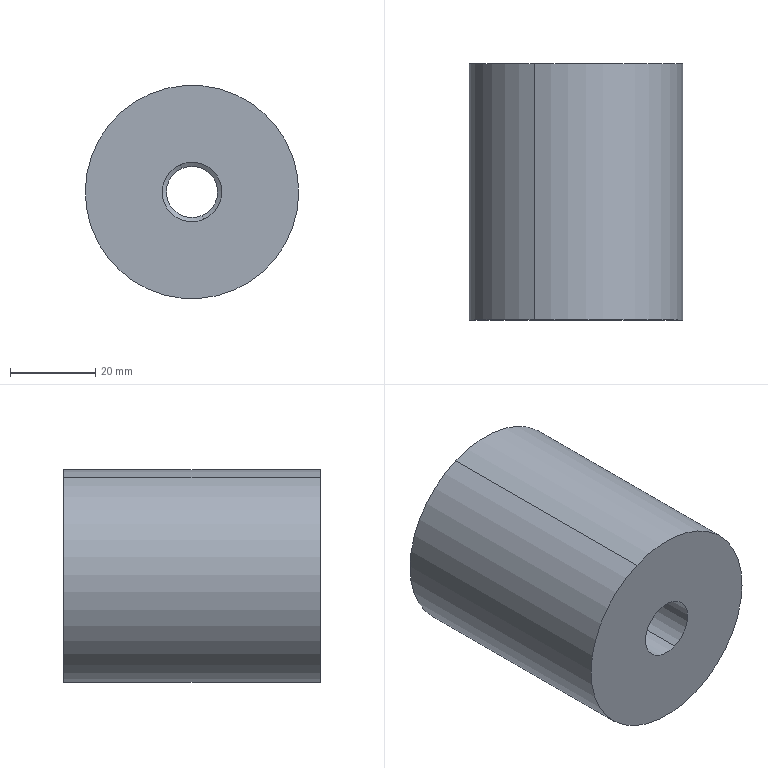Component | SolidWorks | KSD171005A-01-01-22-1 | 1 solid | 10 faces | box 50 x 60 x 50 mm | volume 109378 mm3 | cylinder 6 | cone 2 | plane 2 | commonest cylinder face diameters 14 x2 12 x2 50 x2
build123d program:
from build123d import *

# Parameters (mm, degrees)
SKETCH1_R                      = 25
BOSS_EXTRUDE1_DEPTH            = 60
M12_TAPPED_HOLE1_D             = 12
F_14_0_14_DIAMETER_HOLE1_D     = 14
F_14_0_14_DIAMETER_HOLE1_DEPTH = 40
F_14_0_14_DIAMETER_HOLE1_TIP   = 4.206


with BuildPart() as part:
    # Sketch1 → Boss-Extrude1 (new body)
    with BuildSketch(Plane.XY):
        Circle(SKETCH1_R)
    extrude(amount=BOSS_EXTRUDE1_DEPTH)

    # M12 Tapped Hole1 (through all)
    with Locations(Plane.XY.offset(60)):
        with Locations((0, 0)):
            Hole(M12_TAPPED_HOLE1_D / 2)

    # 14.0 _14_ Diameter Hole1
    with Locations(Plane.XY.offset(60)):
        with Locations((0, 0)):
            Hole(F_14_0_14_DIAMETER_HOLE1_D / 2, depth=F_14_0_14_DIAMETER_HOLE1_DEPTH)
            with Locations((0, 0, -(F_14_0_14_DIAMETER_HOLE1_DEPTH + F_14_0_14_DIAMETER_HOLE1_TIP / 2))):  # 118° drill point
                Cone(0, F_14_0_14_DIAMETER_HOLE1_D / 2, F_14_0_14_DIAMETER_HOLE1_TIP, mode=Mode.SUBTRACT)


solid = part.part

# Placed as in the assembly
solid = solid.moved(Location((-7.111, 170.73, 407), (90, 0, 0)))
STEP:
#1=COLOUR_RGB('',0.7922,0.8196,0.9333);
#2=FILL_AREA_STYLE_COLOUR('',#1);
#3=FILL_AREA_STYLE('',(#2));
#4=SURFACE_STYLE_FILL_AREA(#3);
#5=SURFACE_SIDE_STYLE('',(#4));
#6=SURFACE_STYLE_USAGE(.BOTH.,#5);
#7=PRESENTATION_STYLE_ASSIGNMENT((#6));
#8=CARTESIAN_POINT('',(-0.388,5.934,16.277));
#9=VERTEX_POINT('',#8);
#10=CARTESIAN_POINT('',(-0.172,5.934,15.77));
#11=VERTEX_POINT('',#10);
#12=CARTESIAN_POINT('',(-0.28,5.934,16.024));
#13=DIRECTION('',(0.,-1.,-0.));
#14=DIRECTION('',(0.3918,0.,-0.92));
#15=AXIS2_PLACEMENT_3D('',#12,#13,#14);
#16=CIRCLE('',#15,0.2756);
#17=EDGE_CURVE('',#9,#11,#16,.T.);
#18=ORIENTED_EDGE('',*,*,#17,.F.);
#19=CARTESIAN_POINT('',(-0.388,4.359,16.277));
#20=VERTEX_POINT('',#19);
#21=CARTESIAN_POINT('',(-0.388,4.359,16.277));
#22=DIRECTION('',(0.,-1.,-0.));
#23=VECTOR('',#22,39.37);
#24=LINE('',#21,#23);
#25=EDGE_CURVE('',#9,#20,#24,.T.);
#26=ORIENTED_EDGE('',*,*,#25,.T.);
#27=CARTESIAN_POINT('',(-0.172,4.359,15.77));
#28=VERTEX_POINT('',#27);
#29=CARTESIAN_POINT('',(-0.28,4.359,16.024));
#30=DIRECTION('',(0.,-1.,-0.));
#31=DIRECTION('',(0.3918,0.,-0.92));
#32=AXIS2_PLACEMENT_3D('',#29,#30,#31);
#33=CIRCLE('',#32,0.2756);
#34=EDGE_CURVE('',#20,#28,#33,.T.);
#35=ORIENTED_EDGE('',*,*,#34,.T.);
#36=CARTESIAN_POINT('',(-0.172,4.359,15.77));
#37=DIRECTION('',(0.,-1.,-0.));
#38=VECTOR('',#37,39.37);
#39=LINE('',#36,#38);
#40=EDGE_CURVE('',#11,#28,#39,.T.);
#41=ORIENTED_EDGE('',*,*,#40,.F.);
#42=EDGE_LOOP('',(#18,#26,#35,#41));
#43=FACE_OUTER_BOUND('',#42,.T.);
#44=CARTESIAN_POINT('',(-0.28,4.359,16.024));
#45=DIRECTION('',(0.,-1.,-0.));
#46=DIRECTION('',(0.3918,0.,-0.92));
#47=AXIS2_PLACEMENT_3D('',#44,#45,#46);
#48=CYLINDRICAL_SURFACE('',#47,0.2756);
#49=ADVANCED_FACE('',(#43),#48,.F.);
#50=CARTESIAN_POINT('',(-0.3725,5.958,16.241));
#51=VERTEX_POINT('',#50);
#52=CARTESIAN_POINT('',(-0.1874,5.958,15.806));
#53=VERTEX_POINT('',#52);
#54=CARTESIAN_POINT('',(-0.28,5.958,16.024));
#55=DIRECTION('',(0.,-1.,-0.));
#56=DIRECTION('',(0.3918,0.,-0.92));
#57=AXIS2_PLACEMENT_3D('',#54,#55,#56);
#58=CIRCLE('',#57,0.2362);
#59=EDGE_CURVE('',#51,#53,#58,.T.);
#60=ORIENTED_EDGE('',*,*,#59,.F.);
#61=CARTESIAN_POINT('',(-0.388,5.934,16.277));
#62=DIRECTION('',(-0.3359,-0.515,0.7886));
#63=VECTOR('',#62,39.37);
#64=LINE('',#61,#63);
#65=EDGE_CURVE('',#51,#9,#64,.T.);
#66=ORIENTED_EDGE('',*,*,#65,.T.);
#67=ORIENTED_EDGE('',*,*,#17,.T.);
#68=CARTESIAN_POINT('',(-0.172,5.934,15.77));
#69=DIRECTION('',(0.3359,-0.515,-0.7886));
#70=VECTOR('',#69,39.37);
#71=LINE('',#68,#70);
#72=EDGE_CURVE('',#53,#11,#71,.T.);
#73=ORIENTED_EDGE('',*,*,#72,.F.);
#74=EDGE_LOOP('',(#60,#66,#67,#73));
#75=FACE_OUTER_BOUND('',#74,.T.);
#76=CARTESIAN_POINT('',(-0.28,5.934,16.024));
#77=DIRECTION('',(0.,-1.,-0.));
#78=DIRECTION('',(0.3918,0.,-0.92));
#79=AXIS2_PLACEMENT_3D('',#76,#77,#78);
#80=CONICAL_SURFACE('',#79,0.2756,1.03);
#81=ADVANCED_FACE('',(#75),#80,.F.);
#82=CARTESIAN_POINT('',(-0.3725,6.722,16.241));
#83=VERTEX_POINT('',#82);
#84=CARTESIAN_POINT('',(-0.1874,6.722,15.806));
#85=VERTEX_POINT('',#84);
#86=CARTESIAN_POINT('',(-0.28,6.722,16.024));
#87=DIRECTION('',(0.,-1.,-0.));
#88=DIRECTION('',(0.3918,0.,-0.92));
#89=AXIS2_PLACEMENT_3D('',#86,#87,#88);
#90=CIRCLE('',#89,0.2362);
#91=EDGE_CURVE('',#83,#85,#90,.T.);
#92=ORIENTED_EDGE('',*,*,#91,.F.);
#93=CARTESIAN_POINT('',(-0.3725,4.359,16.241));
#94=DIRECTION('',(0.,-1.,-0.));
#95=VECTOR('',#94,39.37);
#96=LINE('',#93,#95);
#97=EDGE_CURVE('',#83,#51,#96,.T.);
#98=ORIENTED_EDGE('',*,*,#97,.T.);
#99=ORIENTED_EDGE('',*,*,#59,.T.);
#100=CARTESIAN_POINT('',(-0.1874,4.359,15.806));
#101=DIRECTION('',(0.,-1.,-0.));
#102=VECTOR('',#101,39.37);
#103=LINE('',#100,#102);
#104=EDGE_CURVE('',#85,#53,#103,.T.);
#105=ORIENTED_EDGE('',*,*,#104,.F.);
#106=EDGE_LOOP('',(#92,#98,#99,#105));
#107=FACE_OUTER_BOUND('',#106,.T.);
#108=CARTESIAN_POINT('',(-0.28,4.359,16.024));
#109=DIRECTION('',(0.,-1.,-0.));
#110=DIRECTION('',(0.3918,0.,-0.92));
#111=AXIS2_PLACEMENT_3D('',#108,#109,#110);
#112=CYLINDRICAL_SURFACE('',#111,0.2362);
#113=ADVANCED_FACE('',(#107),#112,.F.);
#114=CARTESIAN_POINT('',(0.1057,4.359,15.118));
#115=VERTEX_POINT('',#114);
#116=CARTESIAN_POINT('',(-0.6656,4.359,16.929));
#117=VERTEX_POINT('',#116);
#118=CARTESIAN_POINT('',(-0.28,4.359,16.024));
#119=DIRECTION('',(0.,-1.,-0.));
#120=DIRECTION('',(0.3918,0.,-0.92));
#121=AXIS2_PLACEMENT_3D('',#118,#119,#120);
#122=CIRCLE('',#121,0.9843);
#123=EDGE_CURVE('',#115,#117,#122,.T.);
#124=ORIENTED_EDGE('',*,*,#123,.F.);
#125=CARTESIAN_POINT('',(0.1057,6.722,15.118));
#126=VERTEX_POINT('',#125);
#127=CARTESIAN_POINT('',(0.1057,4.359,15.118));
#128=DIRECTION('',(-0.,1.,0.));
#129=VECTOR('',#128,39.37);
#130=LINE('',#127,#129);
#131=EDGE_CURVE('',#115,#126,#130,.T.);
#132=ORIENTED_EDGE('',*,*,#131,.T.);
#133=CARTESIAN_POINT('',(-0.6656,6.722,16.929));
#134=VERTEX_POINT('',#133);
#135=CARTESIAN_POINT('',(-0.28,6.722,16.024));
#136=DIRECTION('',(0.,-1.,-0.));
#137=DIRECTION('',(0.3918,0.,-0.92));
#138=AXIS2_PLACEMENT_3D('',#135,#136,#137);
#139=CIRCLE('',#138,0.9843);
#140=EDGE_CURVE('',#126,#134,#139,.T.);
#141=ORIENTED_EDGE('',*,*,#140,.T.);
#142=CARTESIAN_POINT('',(-0.6656,4.359,16.929));
#143=DIRECTION('',(-0.,1.,0.));
#144=VECTOR('',#143,39.37);
#145=LINE('',#142,#144);
#146=EDGE_CURVE('',#117,#134,#145,.T.);
#147=ORIENTED_EDGE('',*,*,#146,.F.);
#148=EDGE_LOOP('',(#124,#132,#141,#147));
#149=FACE_OUTER_BOUND('',#148,.T.);
#150=CARTESIAN_POINT('',(-0.28,4.359,16.024));
#151=DIRECTION('',(-0.,1.,0.));
#152=DIRECTION('',(-0.3918,0.,0.92));
#153=AXIS2_PLACEMENT_3D('',#150,#151,#152);
#154=CYLINDRICAL_SURFACE('',#153,0.9843);
#155=ADVANCED_FACE('',(#149),#154,.T.);
#156=ORIENTED_EDGE('',*,*,#131,.F.);
#157=CARTESIAN_POINT('',(-0.28,4.359,16.024));
#158=DIRECTION('',(0.,-1.,-0.));
#159=DIRECTION('',(0.3918,0.,-0.92));
#160=AXIS2_PLACEMENT_3D('',#157,#158,#159);
#161=CIRCLE('',#160,0.9843);
#162=EDGE_CURVE('',#117,#115,#161,.T.);
#163=ORIENTED_EDGE('',*,*,#162,.F.);
#164=ORIENTED_EDGE('',*,*,#146,.T.);
#165=CARTESIAN_POINT('',(-0.28,6.722,16.024));
#166=DIRECTION('',(0.,-1.,-0.));
#167=DIRECTION('',(0.3918,0.,-0.92));
#168=AXIS2_PLACEMENT_3D('',#165,#166,#167);
#169=CIRCLE('',#168,0.9843);
#170=EDGE_CURVE('',#134,#126,#169,.T.);
#171=ORIENTED_EDGE('',*,*,#170,.T.);
#172=EDGE_LOOP('',(#156,#163,#164,#171));
#173=FACE_OUTER_BOUND('',#172,.T.);
#174=CARTESIAN_POINT('',(-0.28,4.359,16.024));
#175=DIRECTION('',(-0.,1.,0.));
#176=DIRECTION('',(-0.3918,0.,0.92));
#177=AXIS2_PLACEMENT_3D('',#174,#175,#176);
#178=CYLINDRICAL_SURFACE('',#177,0.9843);
#179=ADVANCED_FACE('',(#173),#178,.T.);
#180=CARTESIAN_POINT('',(-0.28,4.359,16.024));
#181=DIRECTION('',(0.,-1.,-0.));
#182=DIRECTION('',(0.3918,0.,-0.92));
#183=AXIS2_PLACEMENT_3D('',#180,#181,#182);
#184=CIRCLE('',#183,0.2756);
#185=EDGE_CURVE('',#28,#20,#184,.T.);
#186=ORIENTED_EDGE('',*,*,#185,.F.);
#187=ORIENTED_EDGE('',*,*,#34,.F.);
#188=EDGE_LOOP('',(#186,#187));
#189=FACE_BOUND('',#188,.T.);
#190=ORIENTED_EDGE('',*,*,#162,.T.);
#191=ORIENTED_EDGE('',*,*,#123,.T.);
#192=EDGE_LOOP('',(#190,#191));
#193=FACE_OUTER_BOUND('',#192,.T.);
#194=CARTESIAN_POINT('',(-0.28,4.359,16.024));
#195=DIRECTION('',(0.,-1.,-0.));
#196=DIRECTION('',(0.3918,0.,-0.92));
#197=AXIS2_PLACEMENT_3D('',#194,#195,#196);
#198=PLANE('',#197);
#199=ADVANCED_FACE('',(#189,#193),#198,.T.);
#200=CARTESIAN_POINT('',(-0.28,6.722,16.024));
#201=DIRECTION('',(0.,-1.,-0.));
#202=DIRECTION('',(0.3918,0.,-0.92));
#203=AXIS2_PLACEMENT_3D('',#200,#201,#202);
#204=CIRCLE('',#203,0.2362);
#205=EDGE_CURVE('',#85,#83,#204,.T.);
#206=ORIENTED_EDGE('',*,*,#205,.T.);
#207=ORIENTED_EDGE('',*,*,#91,.T.);
#208=EDGE_LOOP('',(#206,#207));
#209=FACE_BOUND('',#208,.T.);
#210=ORIENTED_EDGE('',*,*,#170,.F.);
#211=ORIENTED_EDGE('',*,*,#140,.F.);
#212=EDGE_LOOP('',(#210,#211));
#213=FACE_OUTER_BOUND('',#212,.T.);
#214=CARTESIAN_POINT('',(-0.28,6.722,16.024));
#215=DIRECTION('',(0.,-1.,-0.));
#216=DIRECTION('',(0.3918,0.,-0.92));
#217=AXIS2_PLACEMENT_3D('',#214,#215,#216);
#218=PLANE('',#217);
#219=ADVANCED_FACE('',(#209,#213),#218,.F.);
#220=ORIENTED_EDGE('',*,*,#97,.F.);
#221=ORIENTED_EDGE('',*,*,#205,.F.);
#222=ORIENTED_EDGE('',*,*,#104,.T.);
#223=CARTESIAN_POINT('',(-0.28,5.958,16.024));
#224=DIRECTION('',(0.,-1.,-0.));
#225=DIRECTION('',(0.3918,0.,-0.92));
#226=AXIS2_PLACEMENT_3D('',#223,#224,#225);
#227=CIRCLE('',#226,0.2362);
#228=EDGE_CURVE('',#53,#51,#227,.T.);
#229=ORIENTED_EDGE('',*,*,#228,.T.);
#230=EDGE_LOOP('',(#220,#221,#222,#229));
#231=FACE_OUTER_BOUND('',#230,.T.);
#232=CARTESIAN_POINT('',(-0.28,4.359,16.024));
#233=DIRECTION('',(0.,-1.,-0.));
#234=DIRECTION('',(0.3918,0.,-0.92));
#235=AXIS2_PLACEMENT_3D('',#232,#233,#234);
#236=CYLINDRICAL_SURFACE('',#235,0.2362);
#237=ADVANCED_FACE('',(#231),#236,.F.);
#238=ORIENTED_EDGE('',*,*,#65,.F.);
#239=ORIENTED_EDGE('',*,*,#228,.F.);
#240=ORIENTED_EDGE('',*,*,#72,.T.);
#241=CARTESIAN_POINT('',(-0.28,5.934,16.024));
#242=DIRECTION('',(0.,-1.,-0.));
#243=DIRECTION('',(0.3918,0.,-0.92));
#244=AXIS2_PLACEMENT_3D('',#241,#242,#243);
#245=CIRCLE('',#244,0.2756);
#246=EDGE_CURVE('',#11,#9,#245,.T.);
#247=ORIENTED_EDGE('',*,*,#246,.T.);
#248=EDGE_LOOP('',(#238,#239,#240,#247));
#249=FACE_OUTER_BOUND('',#248,.T.);
#250=CARTESIAN_POINT('',(-0.28,5.934,16.024));
#251=DIRECTION('',(0.,-1.,-0.));
#252=DIRECTION('',(0.3918,0.,-0.92));
#253=AXIS2_PLACEMENT_3D('',#250,#251,#252);
#254=CONICAL_SURFACE('',#253,0.2756,1.03);
#255=ADVANCED_FACE('',(#249),#254,.F.);
#256=ORIENTED_EDGE('',*,*,#25,.F.);
#257=ORIENTED_EDGE('',*,*,#246,.F.);
#258=ORIENTED_EDGE('',*,*,#40,.T.);
#259=ORIENTED_EDGE('',*,*,#185,.T.);
#260=EDGE_LOOP('',(#256,#257,#258,#259));
#261=FACE_OUTER_BOUND('',#260,.T.);
#262=CARTESIAN_POINT('',(-0.28,4.359,16.024));
#263=DIRECTION('',(0.,-1.,-0.));
#264=DIRECTION('',(0.3918,0.,-0.92));
#265=AXIS2_PLACEMENT_3D('',#262,#263,#264);
#266=CYLINDRICAL_SURFACE('',#265,0.2756);
#267=ADVANCED_FACE('',(#261),#266,.F.);
#268=CLOSED_SHELL('',(#49,#81,#113,#155,#179,#199,#219,#237,#255,#267));
#269=MANIFOLD_SOLID_BREP('',#268);
#270=STYLED_ITEM('',(#7),#269);
#271=PRESENTATION_LAYER_ASSIGNMENT('','',(#270));
#272=CARTESIAN_POINT('',(0.,0.,0.));
#273=DIRECTION('',(0.,0.,1.));
#274=DIRECTION('',(1.,0.,0.));
#275=AXIS2_PLACEMENT_3D('',#272,#273,#274);
#276=(LENGTH_UNIT()NAMED_UNIT(*)SI_UNIT($,.METRE.));
#277=LENGTH_MEASURE_WITH_UNIT(LENGTH_MEASURE(0.0254),#276);
#278=DIMENSIONAL_EXPONENTS(1.,0.,0.,0.,0.,0.,0.);
#279=(CONVERSION_BASED_UNIT('',#277)LENGTH_UNIT()NAMED_UNIT(#278));
#280=UNCERTAINTY_MEASURE_WITH_UNIT(LENGTH_MEASURE(0.00001),#279,'','');
#281=(NAMED_UNIT(*)PLANE_ANGLE_UNIT()SI_UNIT($,.RADIAN.));
#282=(NAMED_UNIT(*)SI_UNIT($,.STERADIAN.)SOLID_ANGLE_UNIT());
#283=(GEOMETRIC_REPRESENTATION_CONTEXT(3)GLOBAL_UNCERTAINTY_ASSIGNED_CONTEXT((#280))GLOBAL_UNIT_ASSIGNED_CONTEXT((#279,#281,#282))REPRESENTATION_CONTEXT('',''));
#284=ADVANCED_BREP_SHAPE_REPRESENTATION('',(#269,#275),#283);
#285=(LENGTH_UNIT()NAMED_UNIT(*)SI_UNIT($,.METRE.));
#286=LENGTH_MEASURE_WITH_UNIT(LENGTH_MEASURE(0.0254),#285);
#287=DIMENSIONAL_EXPONENTS(1.,0.,0.,0.,0.,0.,0.);
#288=(CONVERSION_BASED_UNIT('',#286)LENGTH_UNIT()NAMED_UNIT(#287));
#289=UNCERTAINTY_MEASURE_WITH_UNIT(LENGTH_MEASURE(0.00001),#288,'','');
#290=(NAMED_UNIT(*)PLANE_ANGLE_UNIT()SI_UNIT($,.RADIAN.));
#291=(NAMED_UNIT(*)SI_UNIT($,.STERADIAN.)SOLID_ANGLE_UNIT());
#292=(GEOMETRIC_REPRESENTATION_CONTEXT(3)GLOBAL_UNCERTAINTY_ASSIGNED_CONTEXT((#289))GLOBAL_UNIT_ASSIGNED_CONTEXT((#288,#290,#291))REPRESENTATION_CONTEXT('',''));
#293=MECHANICAL_DESIGN_GEOMETRIC_PRESENTATION_REPRESENTATION('',(#270),#292);